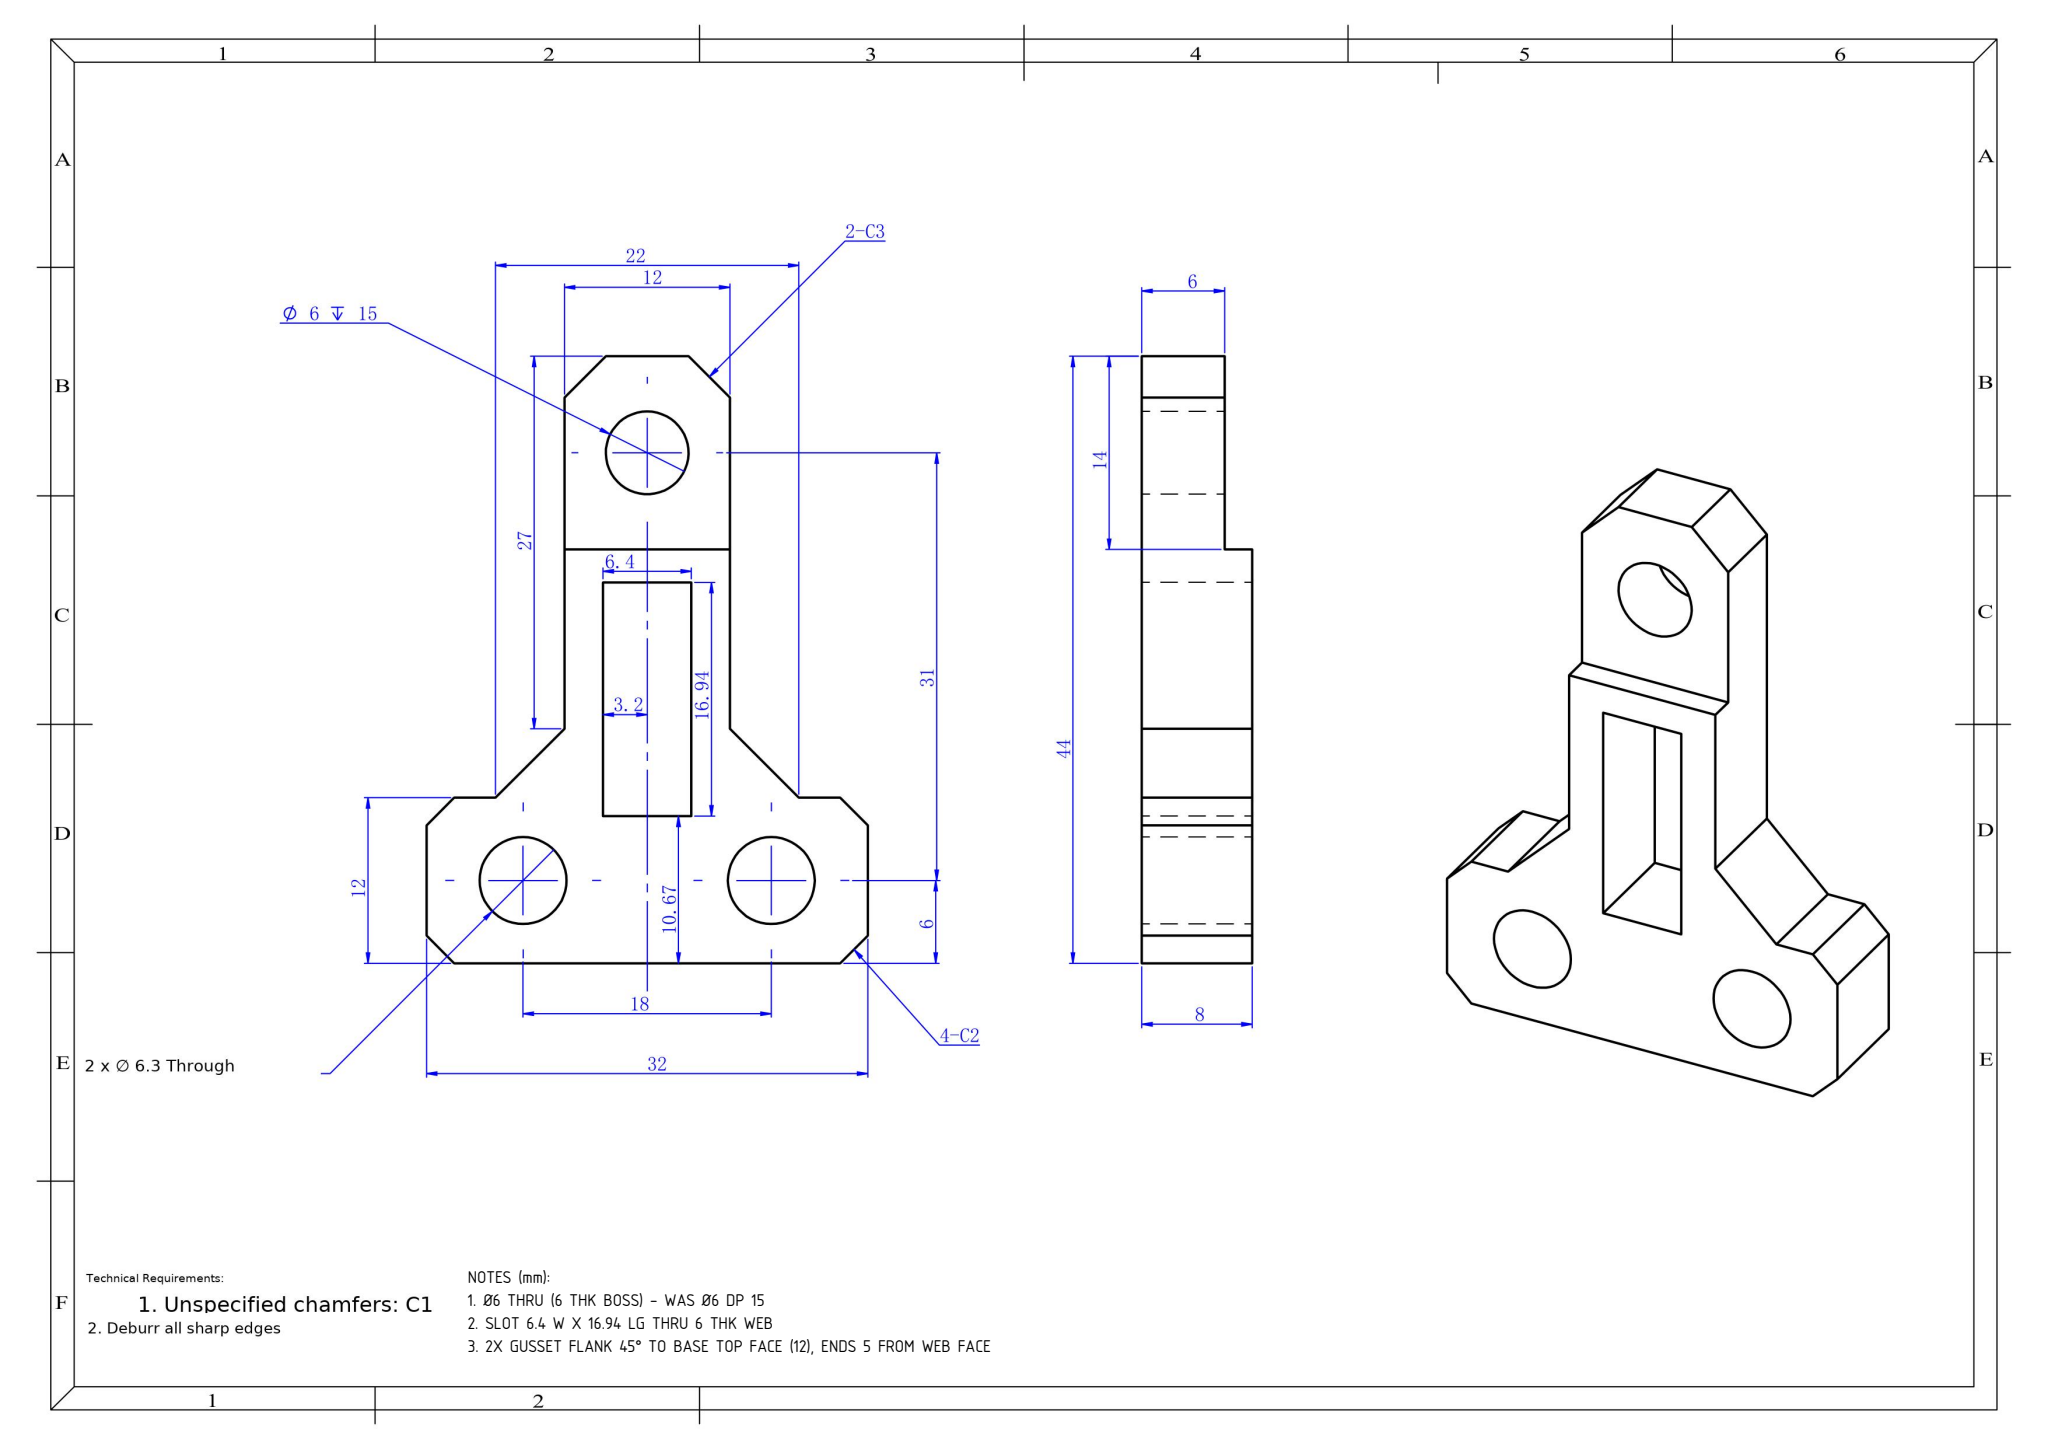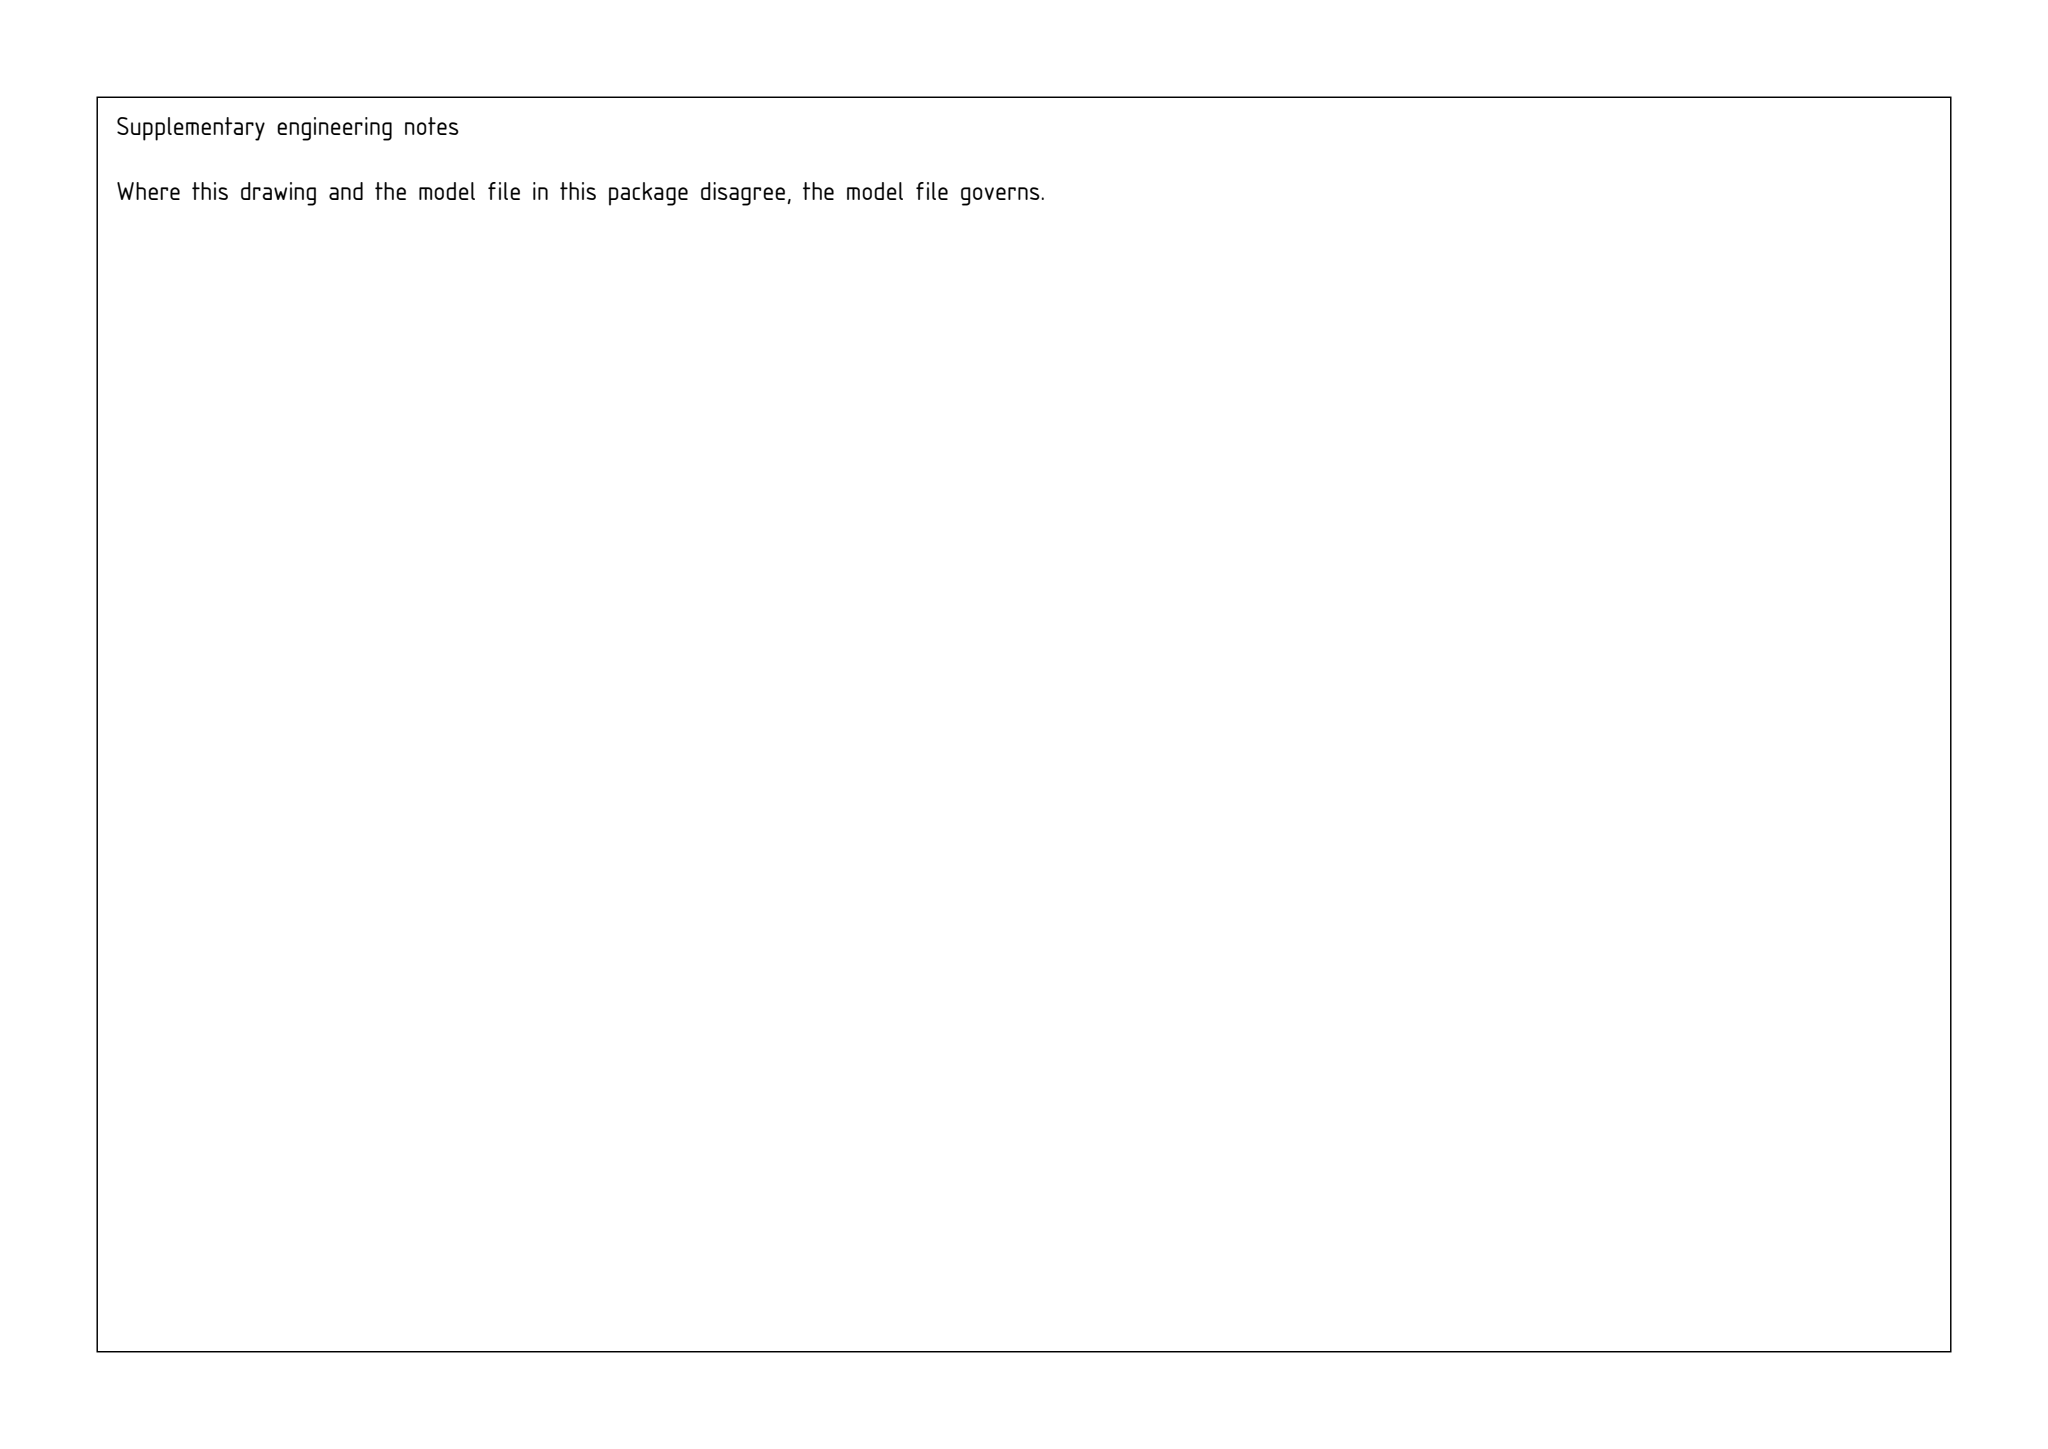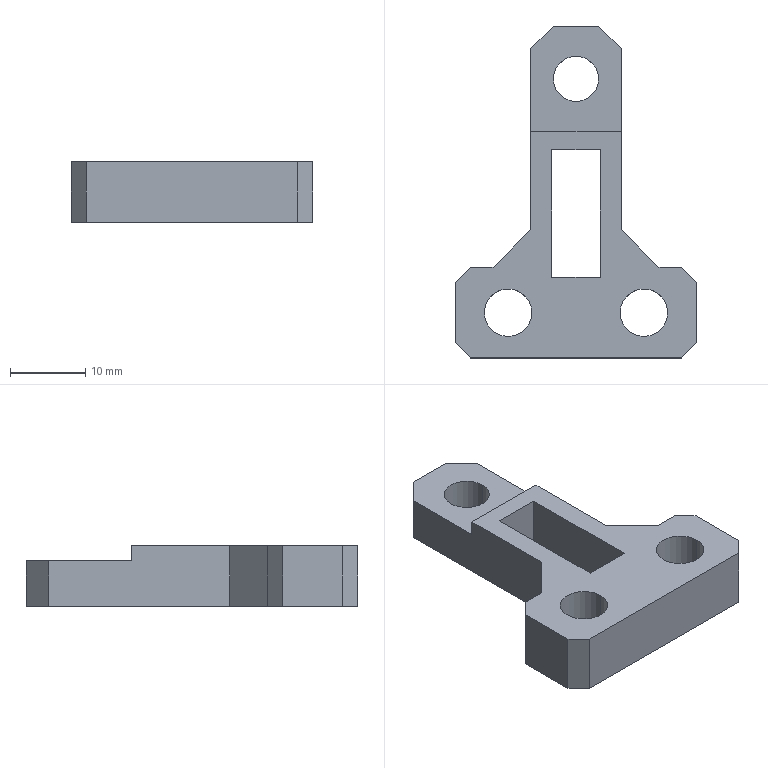Part | SolidWorks | mm | 1 solid | 30 faces | box 32 x 44 x 8 mm | volume 4354 mm3 | plane 24 | cylinder 6 | commonest cylinder face diameters 6.3 x4 6 x2
Drawing notes:
Ø6 THRU (6 THK BOSS) - WAS Ø6 DP 15 | from the solid: cylinder dia 6.0, axis z, length 6.0 at (16,37); z planes only 0/6/8
SLOT 6.4 W X 16.94 LG THRU 6 THK WEB | from the solid: x planes 12.8/19.2 (6.4), y planes 10.67/27.61 (16.94); no z plane between 0 and 6
2X GUSSET FLANK 45° TO BASE TOP FACE (12), ENDS 5 FROM WEB FACE | from the solid: Web faces x=10/22, base top face y=12, flank upper end y=17 (=44-27) on web face, lower ends x=5 & x=27 (22 apart) -> 5 x 5 run/rise = 45 deg
build123d program:
from build123d import *

# Parameters (mm, degrees)
BOSS_EXTRUDE1_DEPTH          = 8
F_6_0_6_DIAMETER_HOLE1_D     = 6
F_6_0_6_DIAMETER_HOLE1_DEPTH = 15
F_6_0_6_DIAMETER_HOLE1_TIP   = 1.803
CUT_EXTRUDE1_DEPTH           = 39.222
CUT_EXTRUDE1_DEPTH_BACK      = 39.222
SKETCH5_W                    = 2
SKETCH5_H                    = 14
CHAMFER1_SIZE                = 3
F_6_3_6_3_DIAMETER_HOLE1_D   = 6.3
CHAMFER2_SIZE                = 2
CHAMFER3_SIZE                = 5
SKETCH8_W                    = 6.398
SKETCH8_H                    = 16.941
CUT_EXTRUDE2_DEPTH           = 18


with BuildPart() as part:
    # Sketch1 → Boss-Extrude1 (new body)
    with BuildSketch(Plane.XY):
        Polygon((-7.233, 13.785), (-7.233, -18.215), (-17.233, -18.215), (-17.233, -30.215), (14.767, -30.215), (14.767, -18.215), (4.767, -18.215), (4.767, 13.785), align=None)
    extrude(amount=BOSS_EXTRUDE1_DEPTH)

    # 6.0 _6_ Diameter Hole1
    with Locations(Plane.XY.offset(8)):
        with Locations((-1.233, 6.785)):
            Hole(F_6_0_6_DIAMETER_HOLE1_D / 2, depth=F_6_0_6_DIAMETER_HOLE1_DEPTH)
            with Locations((0, 0, -(F_6_0_6_DIAMETER_HOLE1_DEPTH + F_6_0_6_DIAMETER_HOLE1_TIP / 2))):  # 118° drill point
                Cone(0, F_6_0_6_DIAMETER_HOLE1_D / 2, F_6_0_6_DIAMETER_HOLE1_TIP, mode=Mode.SUBTRACT)

    # Sketch5 → Cut-Extrude1 (cut, two sides: drawn at the far end of the back side and taken through both)
    with BuildSketch(Plane(origin=(4.767, 0, 0), x_dir=(0, 0, -1), z_dir=(1, 0, 0)).offset(-CUT_EXTRUDE1_DEPTH_BACK)):
        with Locations((-7, 6.785)):
            Rectangle(SKETCH5_W, SKETCH5_H)
    extrude(amount=CUT_EXTRUDE1_DEPTH + CUT_EXTRUDE1_DEPTH_BACK, mode=Mode.SUBTRACT)

    # Chamfer1
    chamfer1_edges = [part.edges().sort_by_distance(p)[0] for p in [
        (-7.233, 13.785, 3),
        (4.767, 13.785, 3),
    ]]
    chamfer(chamfer1_edges, length=CHAMFER1_SIZE)

    # 6.3 _6.3_ Diameter Hole1 (through all)
    with Locations(Plane.XY.offset(8)):
        with Locations((-10.233, -24.215), (7.767, -24.215)):
            Hole(F_6_3_6_3_DIAMETER_HOLE1_D / 2)

    # Chamfer2
    chamfer2_edges = [part.edges().sort_by_distance(p)[0] for p in [
        (14.767, -18.215, 4),
        (14.767, -30.215, 4),
        (-17.233, -30.215, 4),
        (-17.233, -18.215, 4),
    ]]
    chamfer(chamfer2_edges, length=CHAMFER2_SIZE)

    # Chamfer3
    chamfer3_edges = [part.edges().sort_by_distance(p)[0] for p in [
        (-7.233, -18.215, 4),
        (4.767, -18.215, 4),
    ]]
    chamfer(chamfer3_edges, length=CHAMFER3_SIZE)

    # Sketch8 → Cut-Extrude2 (cut)
    with BuildSketch(Plane(origin=(0, 0, 0), x_dir=(-1, 0, 0), z_dir=(0, 0, -1))):
        with Locations((1.233, -11.076)):
            Rectangle(SKETCH8_W, SKETCH8_H)
    extrude(amount=-CUT_EXTRUDE2_DEPTH, mode=Mode.SUBTRACT)


solid = part.part